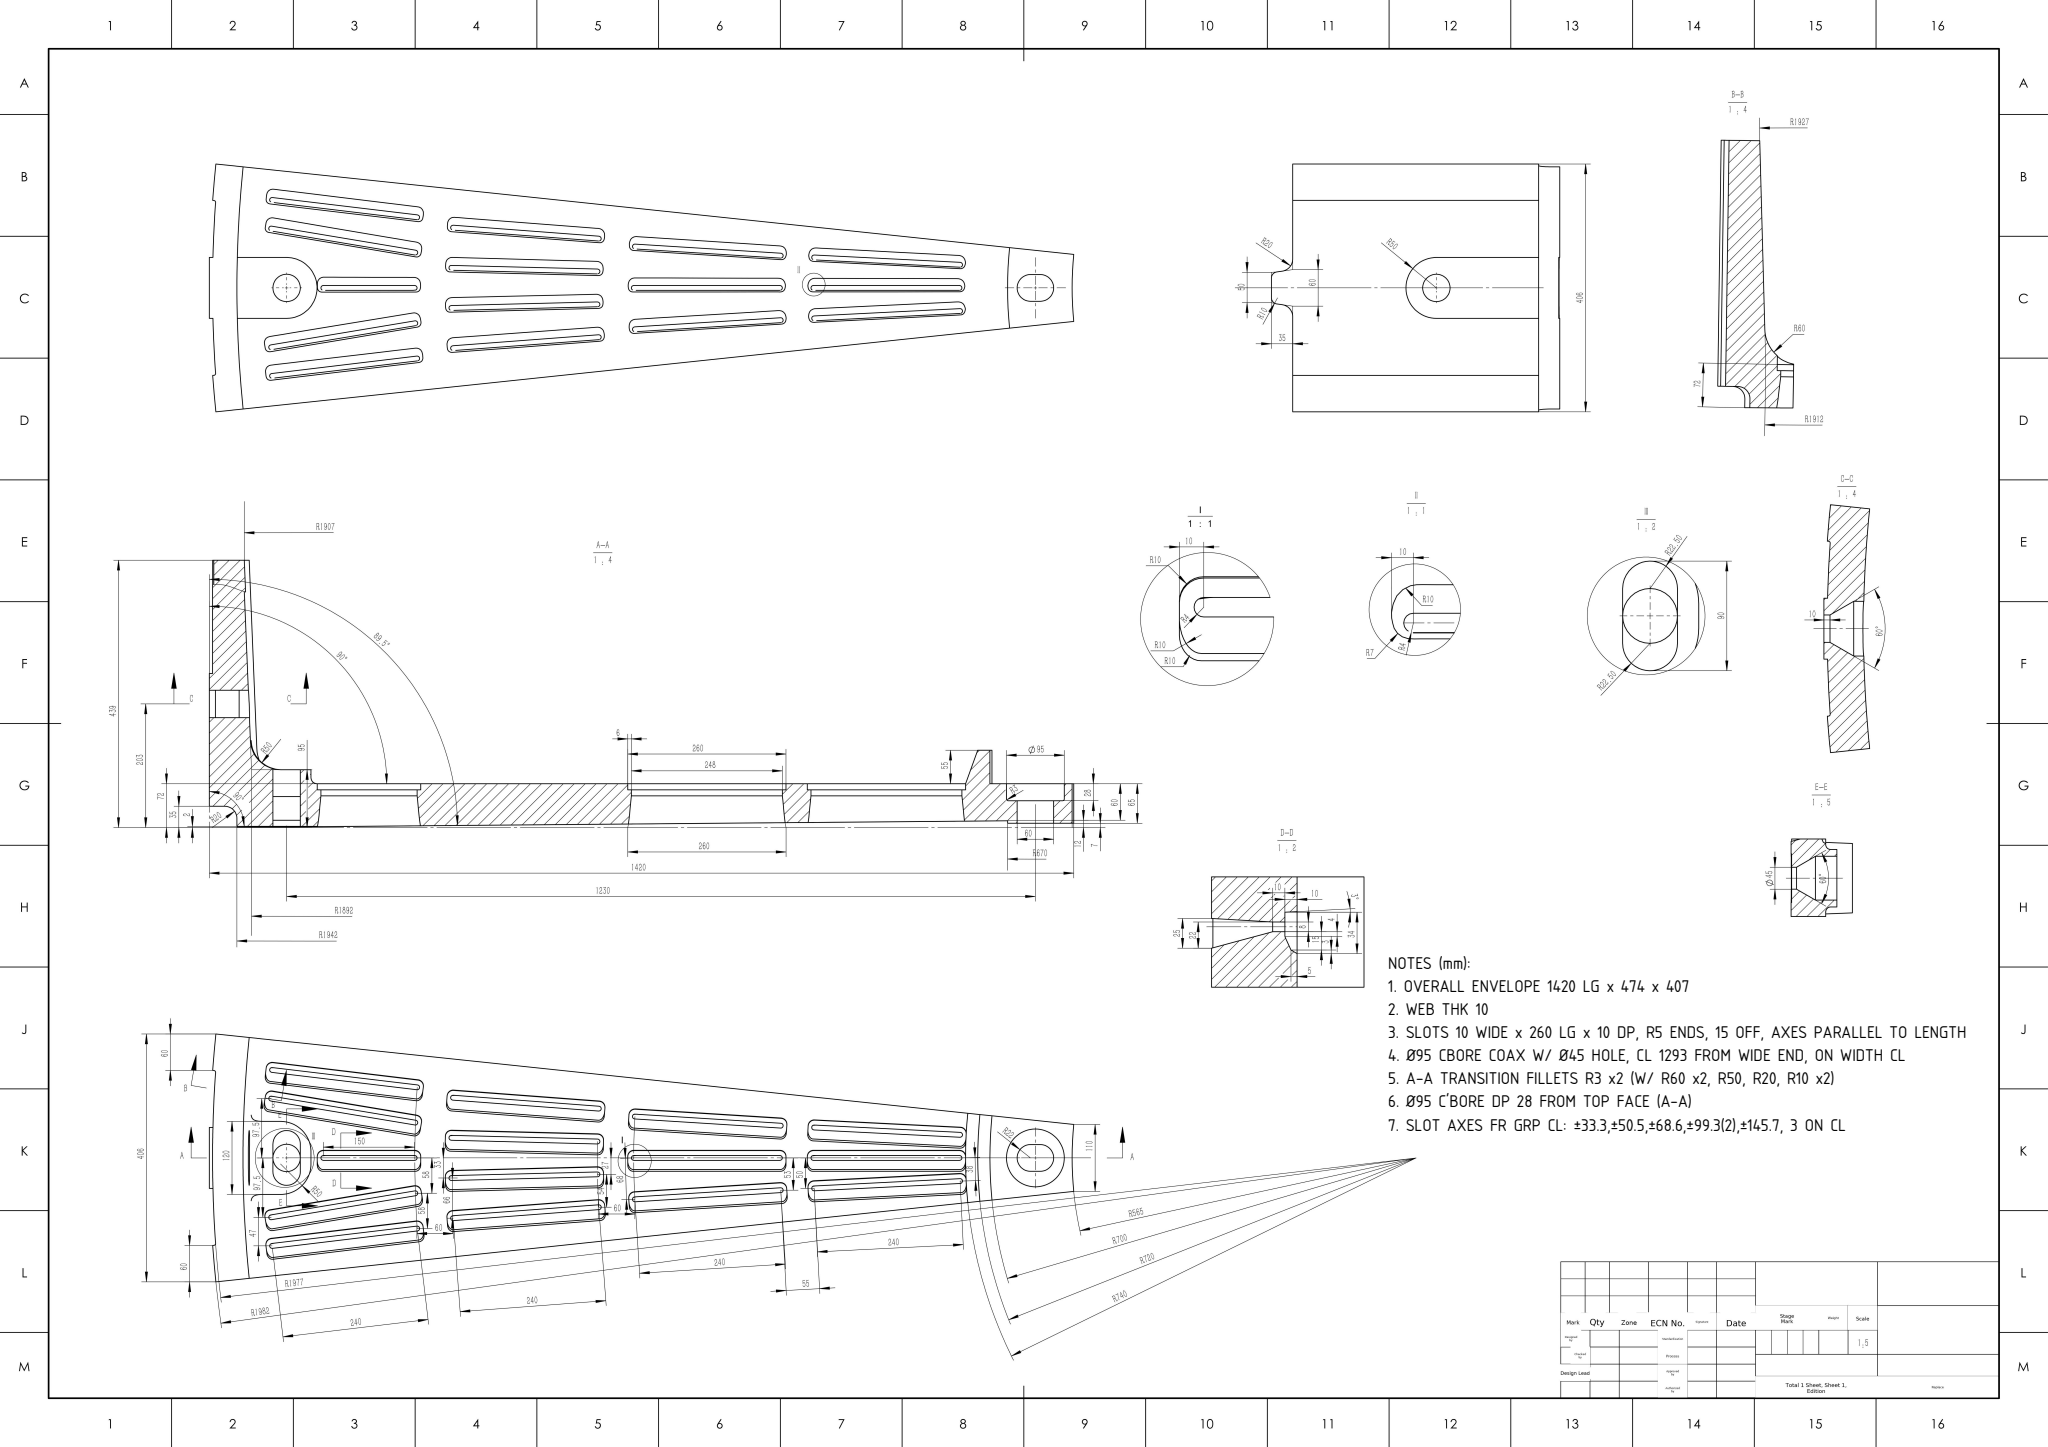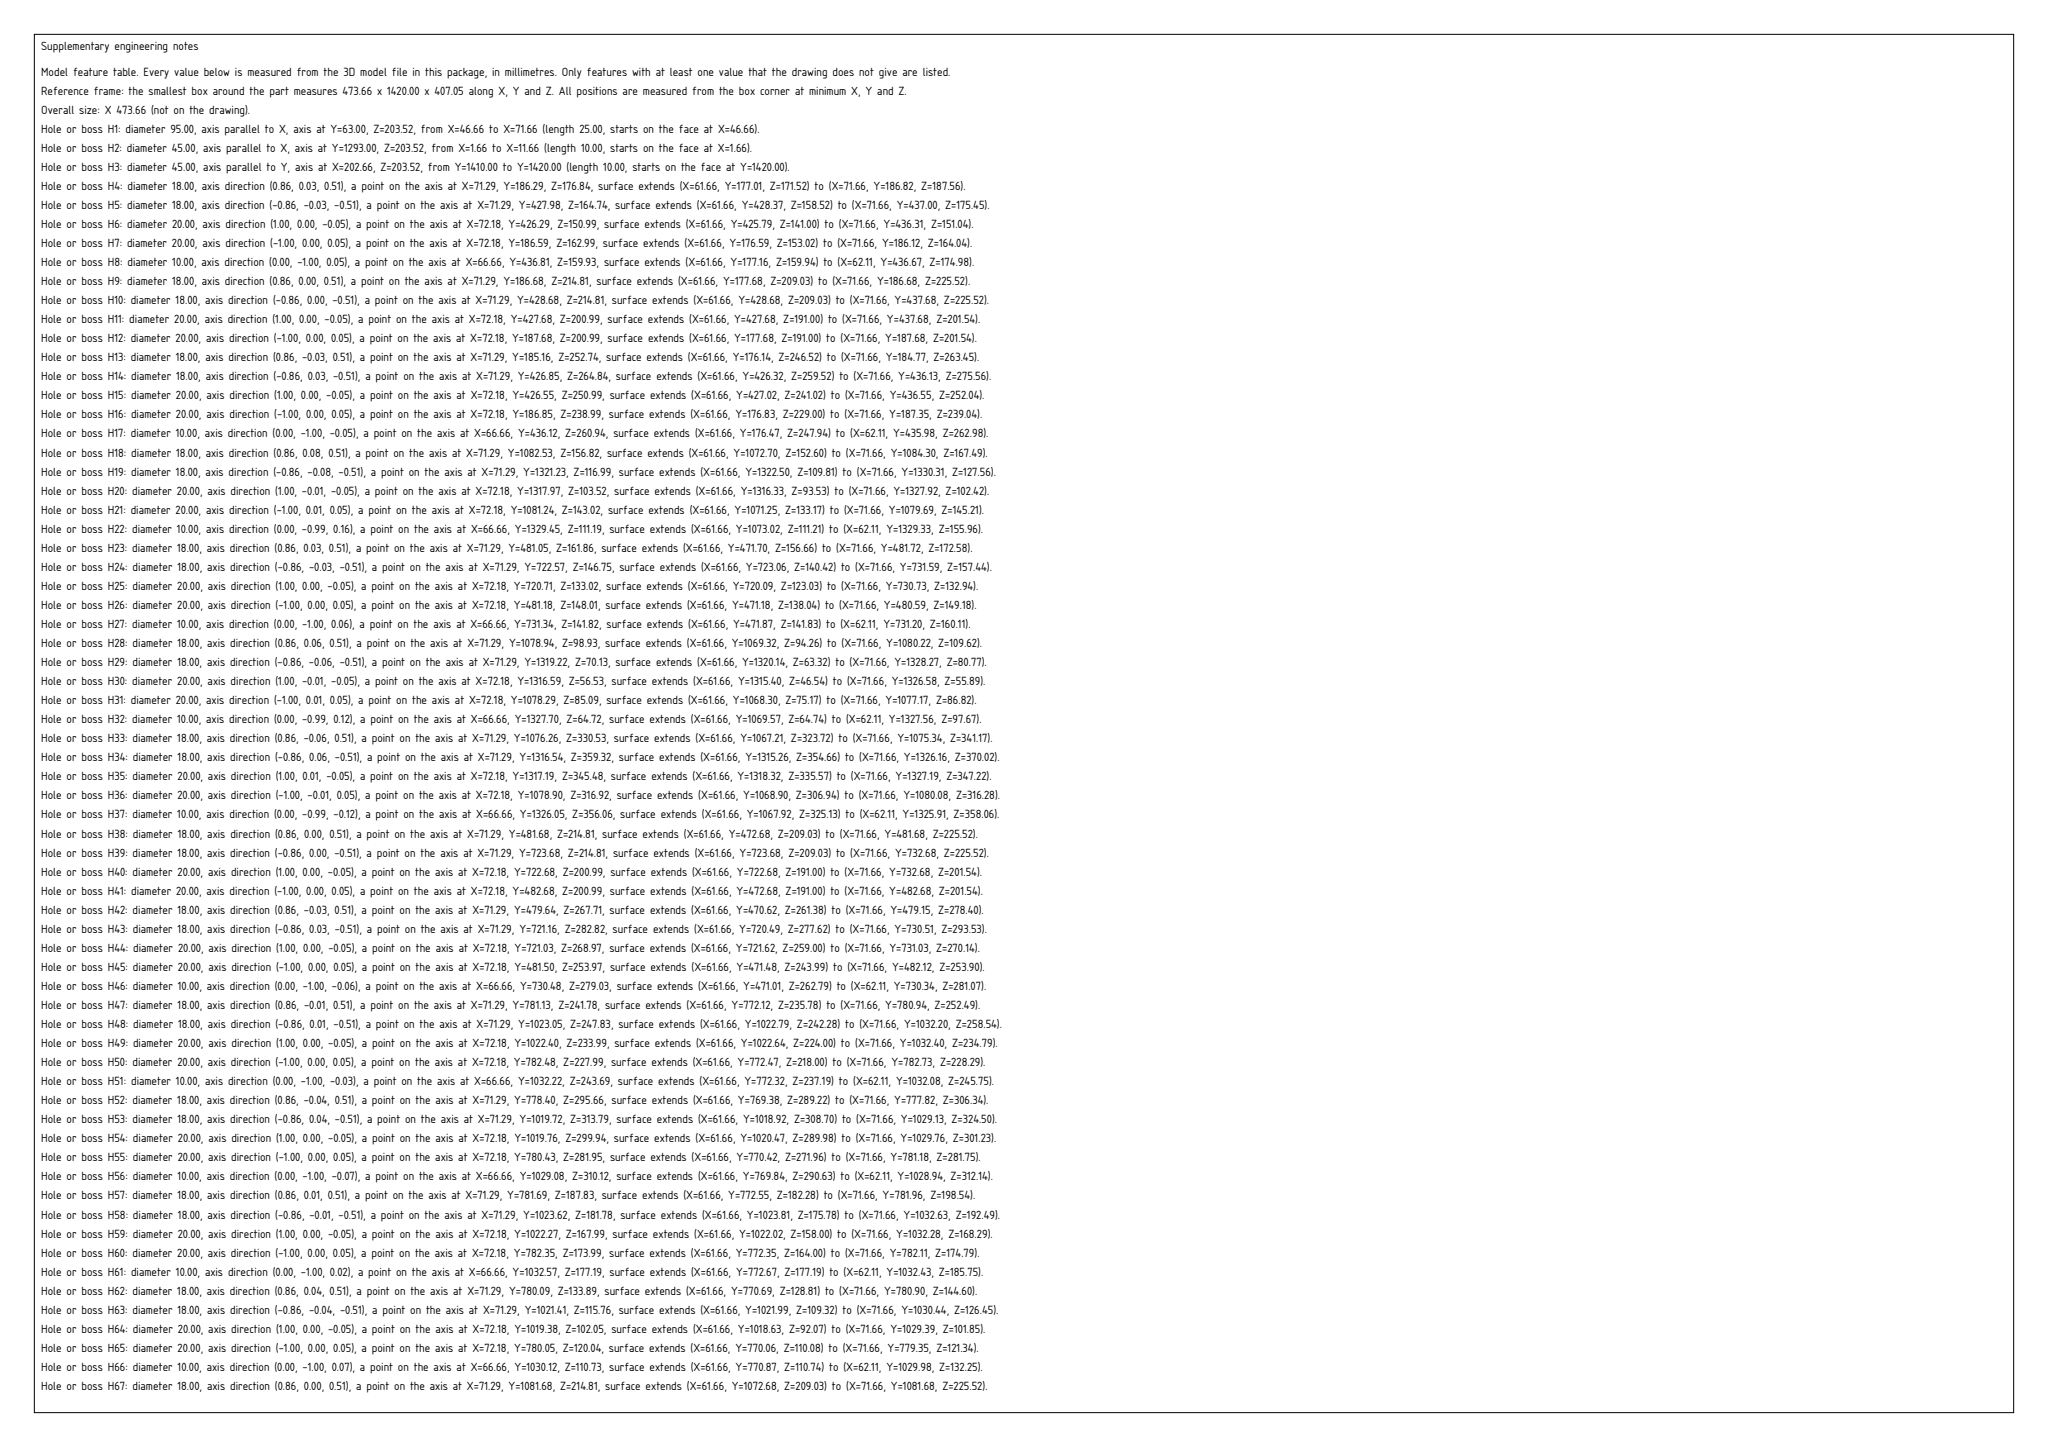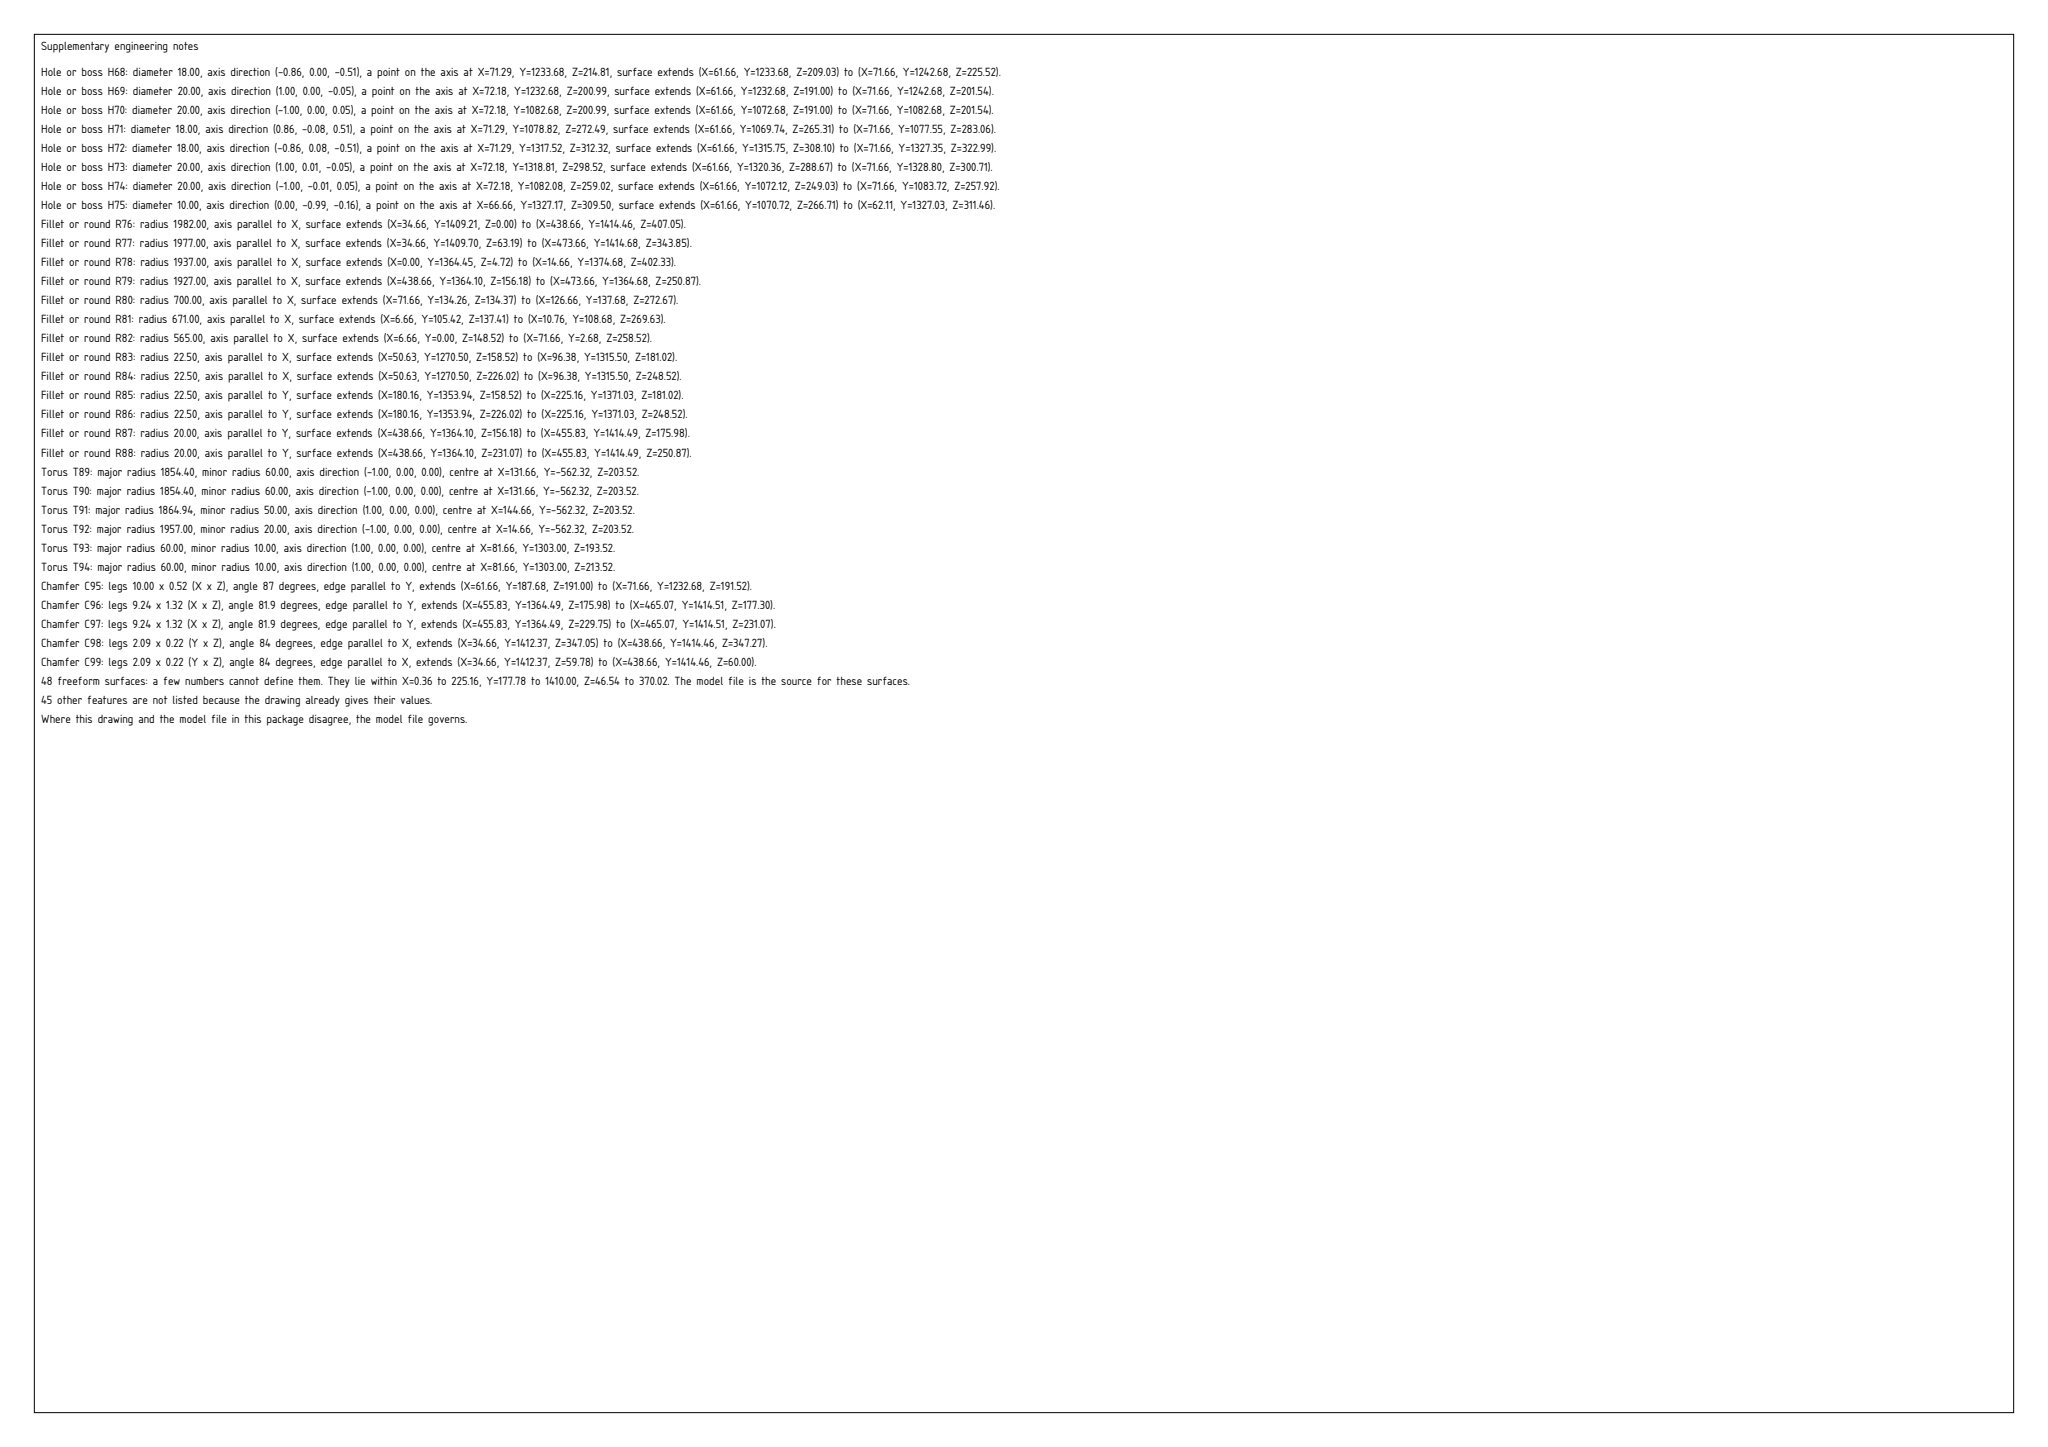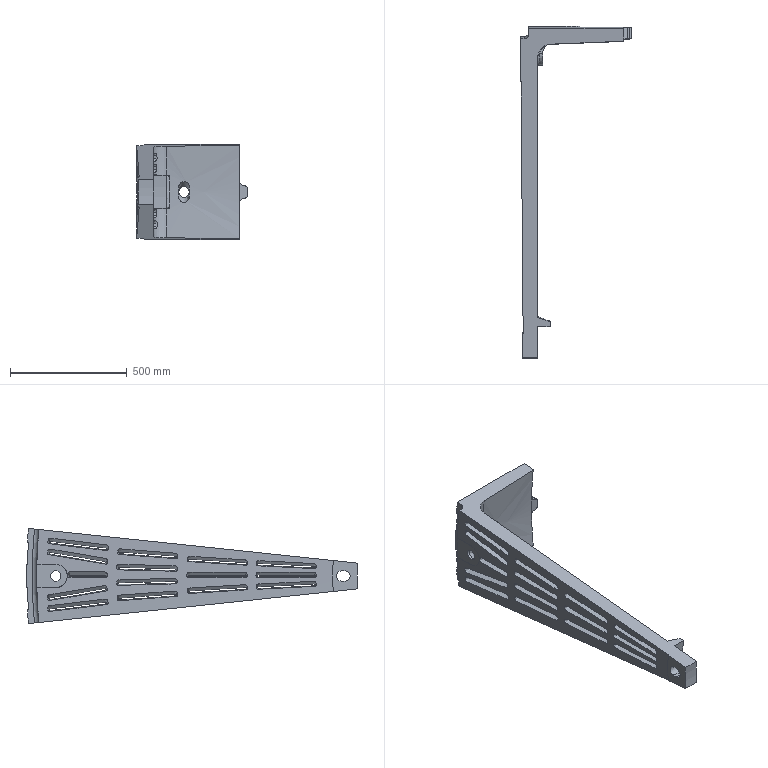Part | SolidWorks | mm | 1 solid | 356 faces | box 473.66 x 1420 x 407.05 mm | volume 28731388 mm3 | plane 159 | cylinder 138 | spline 48 | torus 8 | cone 3 | commonest cylinder face diameters 20 x33 8 x30 18 x30 10 x15 45 x10 100 x4 95 x2 3964 x2
Drawing notes:
OVERALL ENVELOPE 1420 LG x 474 x 407 | from the solid: bbox_xyz [474.001, 1420.005, 407.049]
WEB THK 10 | from the solid: x planes at 62 and 72 give 10 web thk
SLOTS 10 WIDE x 260 LG x 10 DP, R5 ENDS, 15 OFF, AXES PARALLEL TO LENGTH | from the solid: Ø10 cyls axis y at x=67 (web x62-72), lengths 256.6-259.8 (~260); x=62 plane count 15
Ø95 CBORE COAX W/ Ø45 HOLE, CL 1293 FROM WIDE END, ON WIDTH CL | from the solid: tangent planes y=1270.5/1315.5 (Ø45, CL y=1293), z=181.52/225.52 abt width CL z=203.52
A-A TRANSITION FILLETS R3 x2 (W/ R60 x2, R50, R20, R10 x2) | from the solid: fillet_radii [3x2, 60x2, 50, 20, 10x2]
Ø95 C'BORE DP 28 FROM TOP FACE (A-A) | from the solid: x-normal planes at 72.0 and 44.0 (and 35.0/7.0) bound the Ø95 recess: 72-44 = 28 deep
SLOT AXES FR GRP CL: ±33.3,±50.5,±68.6,±99.3(2),±145.7, 3 ON CL | from the solid: 15 dia-10 y-axis slot cylinders at x=67, z = 64.72,110.73,111.19,141.82,159.93,177.19,210.44(x3),243.69,260.94,279.03,309.50,310.12,356.07; symmetric about z=210.44